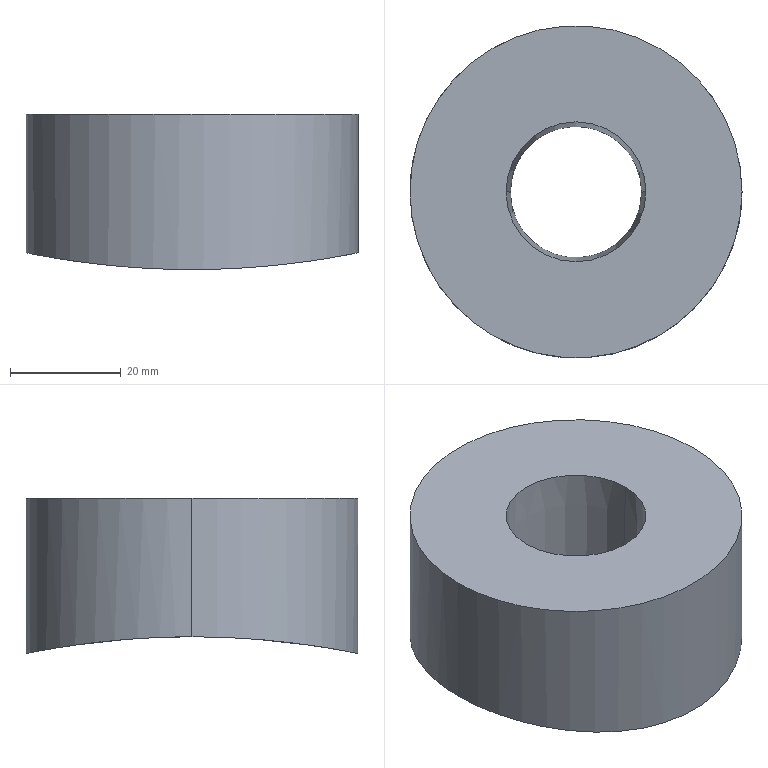Component | SolidWorks | JF21-80.1-1-3(_)-1-SOLID14-1 | 1 solid | 7 faces | box 60 x 60 x 28.03 mm | volume 60972 mm3 | cylinder 4 | cone 2 | plane 1 | commonest cylinder face diameters 300 x2 60 x2
STEP:
#1=COLOUR_RGB('',0.7922,0.8196,0.9333);
#2=FILL_AREA_STYLE_COLOUR('',#1);
#3=FILL_AREA_STYLE('',(#2));
#4=SURFACE_STYLE_FILL_AREA(#3);
#5=SURFACE_SIDE_STYLE('',(#4));
#6=SURFACE_STYLE_USAGE(.BOTH.,#5);
#7=PRESENTATION_STYLE_ASSIGNMENT((#6));
#8=CARTESIAN_POINT('',(11.417,-39.37,42.126));
#9=VERTEX_POINT('',#8);
#10=CARTESIAN_POINT('',(13.78,-39.37,42.126));
#11=VERTEX_POINT('',#10);
#12=CARTESIAN_POINT('',(11.417,-39.37,42.126));
#13=CARTESIAN_POINT('',(11.417,-39.448,42.126));
#14=CARTESIAN_POINT('',(11.425,-39.525,42.124));
#15=CARTESIAN_POINT('',(11.448,-39.639,42.12));
#16=CARTESIAN_POINT('',(11.457,-39.676,42.118));
#17=CARTESIAN_POINT('',(11.474,-39.732,42.115));
#18=CARTESIAN_POINT('',(11.48,-39.75,42.114));
#19=CARTESIAN_POINT('',(11.493,-39.787,42.111));
#20=CARTESIAN_POINT('',(11.5,-39.805,42.11));
#21=CARTESIAN_POINT('',(11.537,-39.894,42.103));
#22=CARTESIAN_POINT('',(11.574,-39.962,42.097));
#23=CARTESIAN_POINT('',(11.627,-40.042,42.088));
#24=CARTESIAN_POINT('',(11.638,-40.058,42.086));
#25=CARTESIAN_POINT('',(11.661,-40.089,42.082));
#26=CARTESIAN_POINT('',(11.673,-40.105,42.08));
#27=CARTESIAN_POINT('',(11.71,-40.15,42.074));
#28=CARTESIAN_POINT('',(11.736,-40.178,42.071));
#29=CARTESIAN_POINT('',(11.818,-40.26,42.059));
#30=CARTESIAN_POINT('',(11.877,-40.308,42.051));
#31=CARTESIAN_POINT('',(11.958,-40.362,42.042));
#32=CARTESIAN_POINT('',(11.974,-40.373,42.04));
#33=CARTESIAN_POINT('',(12.007,-40.393,42.037));
#34=CARTESIAN_POINT('',(12.024,-40.402,42.035));
#35=CARTESIAN_POINT('',(12.075,-40.43,42.03));
#36=CARTESIAN_POINT('',(12.11,-40.446,42.027));
#37=CARTESIAN_POINT('',(12.181,-40.476,42.022));
#38=CARTESIAN_POINT('',(12.217,-40.489,42.019));
#39=CARTESIAN_POINT('',(12.273,-40.506,42.016));
#40=CARTESIAN_POINT('',(12.291,-40.511,42.015));
#41=CARTESIAN_POINT('',(12.329,-40.52,42.013));
#42=CARTESIAN_POINT('',(12.348,-40.525,42.012));
#43=CARTESIAN_POINT('',(12.443,-40.544,42.008));
#44=CARTESIAN_POINT('',(12.52,-40.551,42.007));
#45=CARTESIAN_POINT('',(12.636,-40.551,42.007));
#46=CARTESIAN_POINT('',(12.675,-40.549,42.007));
#47=CARTESIAN_POINT('',(12.733,-40.544,42.008));
#48=CARTESIAN_POINT('',(12.753,-40.541,42.009));
#49=CARTESIAN_POINT('',(12.791,-40.536,42.01));
#50=CARTESIAN_POINT('',(12.81,-40.532,42.011));
#51=CARTESIAN_POINT('',(12.905,-40.513,42.014));
#52=CARTESIAN_POINT('',(12.979,-40.491,42.019));
#53=CARTESIAN_POINT('',(13.086,-40.447,42.027));
#54=CARTESIAN_POINT('',(13.121,-40.43,42.03));
#55=CARTESIAN_POINT('',(13.19,-40.393,42.037));
#56=CARTESIAN_POINT('',(13.223,-40.374,42.04));
#57=CARTESIAN_POINT('',(13.286,-40.331,42.047));
#58=CARTESIAN_POINT('',(13.317,-40.308,42.051));
#59=CARTESIAN_POINT('',(13.362,-40.271,42.057));
#60=CARTESIAN_POINT('',(13.377,-40.259,42.059));
#61=CARTESIAN_POINT('',(13.405,-40.233,42.063));
#62=CARTESIAN_POINT('',(13.419,-40.219,42.065));
#63=CARTESIAN_POINT('',(13.488,-40.151,42.074));
#64=CARTESIAN_POINT('',(13.537,-40.091,42.082));
#65=CARTESIAN_POINT('',(13.601,-39.996,42.093));
#66=CARTESIAN_POINT('',(13.621,-39.963,42.096));
#67=CARTESIAN_POINT('',(13.648,-39.911,42.101));
#68=CARTESIAN_POINT('',(13.657,-39.894,42.103));
#69=CARTESIAN_POINT('',(13.674,-39.859,42.106));
#70=CARTESIAN_POINT('',(13.682,-39.841,42.107));
#71=CARTESIAN_POINT('',(13.719,-39.752,42.114));
#72=CARTESIAN_POINT('',(13.741,-39.678,42.118));
#73=CARTESIAN_POINT('',(13.76,-39.584,42.122));
#74=CARTESIAN_POINT('',(13.764,-39.564,42.123));
#75=CARTESIAN_POINT('',(13.769,-39.526,42.124));
#76=CARTESIAN_POINT('',(13.772,-39.506,42.124));
#77=CARTESIAN_POINT('',(13.778,-39.448,42.126));
#78=CARTESIAN_POINT('',(13.78,-39.409,42.126));
#79=CARTESIAN_POINT('',(13.78,-39.37,42.126));
#80=B_SPLINE_CURVE_WITH_KNOTS('',3,(#12,#13,#14,#15,#16,#17,#18,#19,#20,#21,#22,#23,#24,#25,#26,#27,#28,#29,#30,#31,#32,#33,#34,#35,#36,#37,#38,#39,#40,#41,#42,#43,#44,#45,#46,#47,#48,#49,#50,#51,#52,#53,#54,#55,#56,#57,#58,#59,#60,#61,#62,#63,#64,#65,#66,#67,#68,#69,#70,#71,#72,#73,#74,#75,#76,#77,#78,#79),.UNSPECIFIED.,.F.,.F.,(4,2,2,2,2,2,2,2,2,2,2,2,2,2,2,2,2,2,2,2,2,2,2,2,2,2,2,2,2,2,2,2,2,4),(0.,0.005875,0.008813,0.01028,0.01175,0.01763,0.01909,0.02056,0.0235,0.02938,0.03085,0.03231,0.03525,0.03819,0.03966,0.04113,0.047,0.04994,0.05141,0.05288,0.05875,0.06169,0.06463,0.06757,0.06904,0.0705,0.07638,0.07932,0.08079,0.08226,0.08813,0.0896,0.09107,0.09401),.UNSPECIFIED.);
#81=EDGE_CURVE('',#9,#11,#80,.T.);
#82=ORIENTED_EDGE('',*,*,#81,.F.);
#83=CARTESIAN_POINT('',(12.131,-39.37,42.126));
#84=VERTEX_POINT('',#83);
#85=CARTESIAN_POINT('',(-15.748,-39.37,42.126));
#86=DIRECTION('',(1.,0.,0.));
#87=VECTOR('',#86,39.37);
#88=LINE('',#85,#87);
#89=EDGE_CURVE('',#9,#84,#88,.T.);
#90=ORIENTED_EDGE('',*,*,#89,.T.);
#91=CARTESIAN_POINT('',(13.065,-39.37,42.126));
#92=VERTEX_POINT('',#91);
#93=CARTESIAN_POINT('',(13.065,-39.37,42.126));
#94=CARTESIAN_POINT('',(13.065,-39.401,42.126));
#95=CARTESIAN_POINT('',(13.062,-39.431,42.126));
#96=CARTESIAN_POINT('',(13.053,-39.476,42.125));
#97=CARTESIAN_POINT('',(13.05,-39.491,42.125));
#98=CARTESIAN_POINT('',(13.041,-39.52,42.124));
#99=CARTESIAN_POINT('',(13.036,-39.535,42.124));
#100=CARTESIAN_POINT('',(13.018,-39.577,42.122));
#101=CARTESIAN_POINT('',(13.004,-39.604,42.121));
#102=CARTESIAN_POINT('',(12.978,-39.642,42.12));
#103=CARTESIAN_POINT('',(12.969,-39.654,42.119));
#104=CARTESIAN_POINT('',(12.95,-39.678,42.118));
#105=CARTESIAN_POINT('',(12.939,-39.689,42.117));
#106=CARTESIAN_POINT('',(12.907,-39.721,42.116));
#107=CARTESIAN_POINT('',(12.883,-39.741,42.114));
#108=CARTESIAN_POINT('',(12.845,-39.766,42.113));
#109=CARTESIAN_POINT('',(12.832,-39.774,42.112));
#110=CARTESIAN_POINT('',(12.805,-39.789,42.111));
#111=CARTESIAN_POINT('',(12.778,-39.802,42.11));
#112=CARTESIAN_POINT('',(12.749,-39.812,42.109));
#113=CARTESIAN_POINT('',(12.72,-39.821,42.109));
#114=CARTESIAN_POINT('',(12.705,-39.825,42.108));
#115=CARTESIAN_POINT('',(12.659,-39.834,42.108));
#116=CARTESIAN_POINT('',(12.629,-39.836,42.108));
#117=CARTESIAN_POINT('',(12.584,-39.837,42.108));
#118=CARTESIAN_POINT('',(12.568,-39.836,42.108));
#119=CARTESIAN_POINT('',(12.538,-39.833,42.108));
#120=CARTESIAN_POINT('',(12.522,-39.831,42.108));
#121=CARTESIAN_POINT('',(12.478,-39.822,42.109));
#122=CARTESIAN_POINT('',(12.448,-39.813,42.109));
#123=CARTESIAN_POINT('',(12.406,-39.795,42.111));
#124=CARTESIAN_POINT('',(12.392,-39.789,42.111));
#125=CARTESIAN_POINT('',(12.365,-39.774,42.112));
#126=CARTESIAN_POINT('',(12.352,-39.767,42.113));
#127=CARTESIAN_POINT('',(12.314,-39.741,42.114));
#128=CARTESIAN_POINT('',(12.29,-39.722,42.116));
#129=CARTESIAN_POINT('',(12.247,-39.678,42.118));
#130=CARTESIAN_POINT('',(12.227,-39.655,42.119));
#131=CARTESIAN_POINT('',(12.202,-39.617,42.121));
#132=CARTESIAN_POINT('',(12.194,-39.604,42.121));
#133=CARTESIAN_POINT('',(12.18,-39.577,42.122));
#134=CARTESIAN_POINT('',(12.173,-39.563,42.123));
#135=CARTESIAN_POINT('',(12.155,-39.521,42.124));
#136=CARTESIAN_POINT('',(12.147,-39.492,42.125));
#137=CARTESIAN_POINT('',(12.135,-39.432,42.126));
#138=CARTESIAN_POINT('',(12.131,-39.401,42.126));
#139=CARTESIAN_POINT('',(12.131,-39.37,42.126));
#140=B_SPLINE_CURVE_WITH_KNOTS('',3,(#93,#94,#95,#96,#97,#98,#99,#100,#101,#102,#103,#104,#105,#106,#107,#108,#109,#110,#111,#112,#113,#114,#115,#116,#117,#118,#119,#120,#121,#122,#123,#124,#125,#126,#127,#128,#129,#130,#131,#132,#133,#134,#135,#136,#137,#138,#139),.UNSPECIFIED.,.F.,.F.,(4,2,2,2,2,2,2,2,2,1,2,2,2,2,2,2,2,2,2,2,2,2,2,4),(0.,0.002317,0.003475,0.004634,0.006951,0.008109,0.009267,0.01158,0.01274,0.0139,0.01506,0.01622,0.01853,0.01969,0.02085,0.02317,0.02433,0.02549,0.0278,0.03012,0.03128,0.03244,0.03475,0.03707),.UNSPECIFIED.);
#141=EDGE_CURVE('',#92,#84,#140,.T.);
#142=ORIENTED_EDGE('',*,*,#141,.F.);
#143=CARTESIAN_POINT('',(-15.748,-39.37,42.126));
#144=DIRECTION('',(1.,0.,0.));
#145=VECTOR('',#144,39.37);
#146=LINE('',#143,#145);
#147=EDGE_CURVE('',#92,#11,#146,.T.);
#148=ORIENTED_EDGE('',*,*,#147,.T.);
#149=EDGE_LOOP('',(#82,#90,#142,#148));
#150=FACE_OUTER_BOUND('',#149,.T.);
#151=CARTESIAN_POINT('',(-15.748,-39.37,36.22));
#152=DIRECTION('',(1.,0.,0.));
#153=DIRECTION('',(0.,0.,1.));
#154=AXIS2_PLACEMENT_3D('',#151,#152,#153);
#155=CYLINDRICAL_SURFACE('',#154,5.906);
#156=ADVANCED_FACE('',(#150),#155,.F.);
#157=ORIENTED_EDGE('',*,*,#141,.T.);
#158=CARTESIAN_POINT('',(12.101,-39.37,43.11));
#159=VERTEX_POINT('',#158);
#160=CARTESIAN_POINT('',(12.101,-39.37,43.11));
#161=DIRECTION('',(-0.0312,0.,0.9995));
#162=VECTOR('',#161,39.37);
#163=LINE('',#160,#162);
#164=EDGE_CURVE('',#84,#159,#163,.T.);
#165=ORIENTED_EDGE('',*,*,#164,.T.);
#166=CARTESIAN_POINT('',(13.096,-39.37,43.11));
#167=VERTEX_POINT('',#166);
#168=CARTESIAN_POINT('',(12.598,-39.37,43.11));
#169=DIRECTION('',(0.,0.,1.));
#170=DIRECTION('',(1.,0.,0.));
#171=AXIS2_PLACEMENT_3D('',#168,#169,#170);
#172=CIRCLE('',#171,0.4977);
#173=EDGE_CURVE('',#159,#167,#172,.T.);
#174=ORIENTED_EDGE('',*,*,#173,.T.);
#175=CARTESIAN_POINT('',(13.096,-39.37,43.11));
#176=DIRECTION('',(0.0312,0.,0.9995));
#177=VECTOR('',#176,39.37);
#178=LINE('',#175,#177);
#179=EDGE_CURVE('',#92,#167,#178,.T.);
#180=ORIENTED_EDGE('',*,*,#179,.F.);
#181=EDGE_LOOP('',(#157,#165,#174,#180));
#182=FACE_OUTER_BOUND('',#181,.T.);
#183=CARTESIAN_POINT('',(12.598,-39.37,43.11));
#184=DIRECTION('',(0.,0.,1.));
#185=DIRECTION('',(-1.,0.,0.));
#186=AXIS2_PLACEMENT_3D('',#183,#184,#185);
#187=CONICAL_SURFACE('',#186,0.4977,0.03121);
#188=ADVANCED_FACE('',(#182),#187,.F.);
#189=CARTESIAN_POINT('',(13.78,-39.37,42.126));
#190=CARTESIAN_POINT('',(13.78,-39.292,42.126));
#191=CARTESIAN_POINT('',(13.772,-39.215,42.124));
#192=CARTESIAN_POINT('',(13.749,-39.102,42.12));
#193=CARTESIAN_POINT('',(13.74,-39.064,42.118));
#194=CARTESIAN_POINT('',(13.723,-39.008,42.115));
#195=CARTESIAN_POINT('',(13.717,-38.99,42.114));
#196=CARTESIAN_POINT('',(13.704,-38.953,42.111));
#197=CARTESIAN_POINT('',(13.697,-38.935,42.11));
#198=CARTESIAN_POINT('',(13.66,-38.846,42.103));
#199=CARTESIAN_POINT('',(13.623,-38.778,42.097));
#200=CARTESIAN_POINT('',(13.57,-38.698,42.088));
#201=CARTESIAN_POINT('',(13.559,-38.682,42.086));
#202=CARTESIAN_POINT('',(13.536,-38.651,42.082));
#203=CARTESIAN_POINT('',(13.524,-38.636,42.08));
#204=CARTESIAN_POINT('',(13.487,-38.591,42.074));
#205=CARTESIAN_POINT('',(13.461,-38.562,42.071));
#206=CARTESIAN_POINT('',(13.379,-38.481,42.059));
#207=CARTESIAN_POINT('',(13.32,-38.432,42.051));
#208=CARTESIAN_POINT('',(13.239,-38.378,42.042));
#209=CARTESIAN_POINT('',(13.223,-38.367,42.04));
#210=CARTESIAN_POINT('',(13.19,-38.347,42.037));
#211=CARTESIAN_POINT('',(13.173,-38.338,42.035));
#212=CARTESIAN_POINT('',(13.122,-38.311,42.03));
#213=CARTESIAN_POINT('',(13.087,-38.294,42.027));
#214=CARTESIAN_POINT('',(13.016,-38.265,42.022));
#215=CARTESIAN_POINT('',(12.98,-38.252,42.019));
#216=CARTESIAN_POINT('',(12.924,-38.235,42.016));
#217=CARTESIAN_POINT('',(12.906,-38.229,42.015));
#218=CARTESIAN_POINT('',(12.868,-38.22,42.013));
#219=CARTESIAN_POINT('',(12.849,-38.216,42.012));
#220=CARTESIAN_POINT('',(12.753,-38.197,42.008));
#221=CARTESIAN_POINT('',(12.677,-38.189,42.007));
#222=CARTESIAN_POINT('',(12.561,-38.189,42.007));
#223=CARTESIAN_POINT('',(12.522,-38.191,42.007));
#224=CARTESIAN_POINT('',(12.464,-38.197,42.008));
#225=CARTESIAN_POINT('',(12.444,-38.199,42.009));
#226=CARTESIAN_POINT('',(12.406,-38.205,42.01));
#227=CARTESIAN_POINT('',(12.387,-38.208,42.011));
#228=CARTESIAN_POINT('',(12.292,-38.227,42.014));
#229=CARTESIAN_POINT('',(12.218,-38.249,42.019));
#230=CARTESIAN_POINT('',(12.111,-38.294,42.027));
#231=CARTESIAN_POINT('',(12.076,-38.31,42.03));
#232=CARTESIAN_POINT('',(12.007,-38.347,42.037));
#233=CARTESIAN_POINT('',(11.974,-38.367,42.04));
#234=CARTESIAN_POINT('',(11.91,-38.409,42.047));
#235=CARTESIAN_POINT('',(11.88,-38.432,42.051));
#236=CARTESIAN_POINT('',(11.835,-38.469,42.057));
#237=CARTESIAN_POINT('',(11.82,-38.481,42.059));
#238=CARTESIAN_POINT('',(11.792,-38.507,42.063));
#239=CARTESIAN_POINT('',(11.777,-38.521,42.065));
#240=CARTESIAN_POINT('',(11.709,-38.589,42.074));
#241=CARTESIAN_POINT('',(11.66,-38.649,42.082));
#242=CARTESIAN_POINT('',(11.596,-38.744,42.093));
#243=CARTESIAN_POINT('',(11.576,-38.777,42.096));
#244=CARTESIAN_POINT('',(11.548,-38.829,42.101));
#245=CARTESIAN_POINT('',(11.54,-38.846,42.103));
#246=CARTESIAN_POINT('',(11.523,-38.881,42.106));
#247=CARTESIAN_POINT('',(11.515,-38.899,42.107));
#248=CARTESIAN_POINT('',(11.478,-38.988,42.114));
#249=CARTESIAN_POINT('',(11.456,-39.062,42.118));
#250=CARTESIAN_POINT('',(11.437,-39.157,42.122));
#251=CARTESIAN_POINT('',(11.433,-39.176,42.123));
#252=CARTESIAN_POINT('',(11.427,-39.214,42.124));
#253=CARTESIAN_POINT('',(11.425,-39.234,42.124));
#254=CARTESIAN_POINT('',(11.419,-39.292,42.126));
#255=CARTESIAN_POINT('',(11.417,-39.331,42.126));
#256=CARTESIAN_POINT('',(11.417,-39.37,42.126));
#257=B_SPLINE_CURVE_WITH_KNOTS('',3,(#189,#190,#191,#192,#193,#194,#195,#196,#197,#198,#199,#200,#201,#202,#203,#204,#205,#206,#207,#208,#209,#210,#211,#212,#213,#214,#215,#216,#217,#218,#219,#220,#221,#222,#223,#224,#225,#226,#227,#228,#229,#230,#231,#232,#233,#234,#235,#236,#237,#238,#239,#240,#241,#242,#243,#244,#245,#246,#247,#248,#249,#250,#251,#252,#253,#254,#255,#256),.UNSPECIFIED.,.F.,.F.,(4,2,2,2,2,2,2,2,2,2,2,2,2,2,2,2,2,2,2,2,2,2,2,2,2,2,2,2,2,2,2,2,2,4),(0.,0.005875,0.008813,0.01028,0.01175,0.01763,0.01909,0.02056,0.0235,0.02938,0.03085,0.03231,0.03525,0.03819,0.03966,0.04113,0.047,0.04994,0.05141,0.05288,0.05875,0.06169,0.06463,0.06757,0.06904,0.0705,0.07638,0.07932,0.08079,0.08226,0.08813,0.0896,0.09107,0.09401),.UNSPECIFIED.);
#258=EDGE_CURVE('',#11,#9,#257,.T.);
#259=ORIENTED_EDGE('',*,*,#258,.T.);
#260=CARTESIAN_POINT('',(11.417,-39.37,43.11));
#261=VERTEX_POINT('',#260);
#262=CARTESIAN_POINT('',(11.417,-39.37,41.929));
#263=DIRECTION('',(0.,0.,1.));
#264=VECTOR('',#263,39.37);
#265=LINE('',#262,#264);
#266=EDGE_CURVE('',#9,#261,#265,.T.);
#267=ORIENTED_EDGE('',*,*,#266,.T.);
#268=CARTESIAN_POINT('',(13.78,-39.37,43.11));
#269=VERTEX_POINT('',#268);
#270=CARTESIAN_POINT('',(12.598,-39.37,43.11));
#271=DIRECTION('',(0.,0.,1.));
#272=DIRECTION('',(1.,0.,0.));
#273=AXIS2_PLACEMENT_3D('',#270,#271,#272);
#274=CIRCLE('',#273,1.181);
#275=EDGE_CURVE('',#269,#261,#274,.T.);
#276=ORIENTED_EDGE('',*,*,#275,.F.);
#277=CARTESIAN_POINT('',(13.78,-39.37,41.929));
#278=DIRECTION('',(0.,0.,1.));
#279=VECTOR('',#278,39.37);
#280=LINE('',#277,#279);
#281=EDGE_CURVE('',#11,#269,#280,.T.);
#282=ORIENTED_EDGE('',*,*,#281,.F.);
#283=EDGE_LOOP('',(#259,#267,#276,#282));
#284=FACE_OUTER_BOUND('',#283,.T.);
#285=CARTESIAN_POINT('',(12.598,-39.37,41.929));
#286=DIRECTION('',(0.,0.,1.));
#287=DIRECTION('',(-1.,0.,0.));
#288=AXIS2_PLACEMENT_3D('',#285,#286,#287);
#289=CYLINDRICAL_SURFACE('',#288,1.181);
#290=ADVANCED_FACE('',(#284),#289,.T.);
#291=ORIENTED_EDGE('',*,*,#266,.F.);
#292=ORIENTED_EDGE('',*,*,#81,.T.);
#293=ORIENTED_EDGE('',*,*,#281,.T.);
#294=CARTESIAN_POINT('',(12.598,-39.37,43.11));
#295=DIRECTION('',(0.,0.,1.));
#296=DIRECTION('',(1.,0.,0.));
#297=AXIS2_PLACEMENT_3D('',#294,#295,#296);
#298=CIRCLE('',#297,1.181);
#299=EDGE_CURVE('',#261,#269,#298,.T.);
#300=ORIENTED_EDGE('',*,*,#299,.F.);
#301=EDGE_LOOP('',(#291,#292,#293,#300));
#302=FACE_OUTER_BOUND('',#301,.T.);
#303=CARTESIAN_POINT('',(12.598,-39.37,41.929));
#304=DIRECTION('',(0.,0.,1.));
#305=DIRECTION('',(-1.,0.,0.));
#306=AXIS2_PLACEMENT_3D('',#303,#304,#305);
#307=CYLINDRICAL_SURFACE('',#306,1.181);
#308=ADVANCED_FACE('',(#302),#307,.T.);
#309=CARTESIAN_POINT('',(12.598,-39.37,43.11));
#310=DIRECTION('',(0.,0.,1.));
#311=DIRECTION('',(1.,0.,0.));
#312=AXIS2_PLACEMENT_3D('',#309,#310,#311);
#313=CIRCLE('',#312,0.4977);
#314=EDGE_CURVE('',#167,#159,#313,.T.);
#315=ORIENTED_EDGE('',*,*,#314,.F.);
#316=ORIENTED_EDGE('',*,*,#173,.F.);
#317=EDGE_LOOP('',(#315,#316));
#318=FACE_BOUND('',#317,.T.);
#319=ORIENTED_EDGE('',*,*,#275,.T.);
#320=ORIENTED_EDGE('',*,*,#299,.T.);
#321=EDGE_LOOP('',(#319,#320));
#322=FACE_OUTER_BOUND('',#321,.T.);
#323=CARTESIAN_POINT('',(12.598,-39.37,43.11));
#324=DIRECTION('',(0.,0.,1.));
#325=DIRECTION('',(-1.,0.,0.));
#326=AXIS2_PLACEMENT_3D('',#323,#324,#325);
#327=PLANE('',#326);
#328=ADVANCED_FACE('',(#318,#322),#327,.T.);
#329=ORIENTED_EDGE('',*,*,#89,.F.);
#330=ORIENTED_EDGE('',*,*,#258,.F.);
#331=ORIENTED_EDGE('',*,*,#147,.F.);
#332=CARTESIAN_POINT('',(12.131,-39.37,42.126));
#333=CARTESIAN_POINT('',(12.131,-39.339,42.126));
#334=CARTESIAN_POINT('',(12.134,-39.309,42.126));
#335=CARTESIAN_POINT('',(12.143,-39.264,42.125));
#336=CARTESIAN_POINT('',(12.147,-39.249,42.125));
#337=CARTESIAN_POINT('',(12.156,-39.22,42.124));
#338=CARTESIAN_POINT('',(12.161,-39.205,42.124));
#339=CARTESIAN_POINT('',(12.179,-39.163,42.122));
#340=CARTESIAN_POINT('',(12.193,-39.136,42.121));
#341=CARTESIAN_POINT('',(12.219,-39.098,42.12));
#342=CARTESIAN_POINT('',(12.228,-39.086,42.119));
#343=CARTESIAN_POINT('',(12.247,-39.062,42.118));
#344=CARTESIAN_POINT('',(12.258,-39.051,42.117));
#345=CARTESIAN_POINT('',(12.29,-39.019,42.116));
#346=CARTESIAN_POINT('',(12.313,-38.999,42.114));
#347=CARTESIAN_POINT('',(12.352,-38.974,42.113));
#348=CARTESIAN_POINT('',(12.365,-38.966,42.112));
#349=CARTESIAN_POINT('',(12.392,-38.951,42.111));
#350=CARTESIAN_POINT('',(12.419,-38.939,42.11));
#351=CARTESIAN_POINT('',(12.448,-38.928,42.109));
#352=CARTESIAN_POINT('',(12.477,-38.919,42.109));
#353=CARTESIAN_POINT('',(12.492,-38.916,42.108));
#354=CARTESIAN_POINT('',(12.537,-38.907,42.108));
#355=CARTESIAN_POINT('',(12.568,-38.904,42.108));
#356=CARTESIAN_POINT('',(12.613,-38.904,42.108));
#357=CARTESIAN_POINT('',(12.629,-38.904,42.108));
#358=CARTESIAN_POINT('',(12.659,-38.907,42.108));
#359=CARTESIAN_POINT('',(12.674,-38.91,42.108));
#360=CARTESIAN_POINT('',(12.719,-38.919,42.109));
#361=CARTESIAN_POINT('',(12.748,-38.927,42.109));
#362=CARTESIAN_POINT('',(12.791,-38.945,42.111));
#363=CARTESIAN_POINT('',(12.805,-38.951,42.111));
#364=CARTESIAN_POINT('',(12.832,-38.966,42.112));
#365=CARTESIAN_POINT('',(12.845,-38.974,42.113));
#366=CARTESIAN_POINT('',(12.883,-38.999,42.114));
#367=CARTESIAN_POINT('',(12.906,-39.018,42.116));
#368=CARTESIAN_POINT('',(12.95,-39.062,42.118));
#369=CARTESIAN_POINT('',(12.969,-39.085,42.119));
#370=CARTESIAN_POINT('',(12.995,-39.123,42.121));
#371=CARTESIAN_POINT('',(13.003,-39.136,42.121));
#372=CARTESIAN_POINT('',(13.017,-39.163,42.122));
#373=CARTESIAN_POINT('',(13.024,-39.177,42.123));
#374=CARTESIAN_POINT('',(13.041,-39.219,42.124));
#375=CARTESIAN_POINT('',(13.05,-39.249,42.125));
#376=CARTESIAN_POINT('',(13.062,-39.308,42.126));
#377=CARTESIAN_POINT('',(13.065,-39.339,42.126));
#378=CARTESIAN_POINT('',(13.065,-39.37,42.126));
#379=B_SPLINE_CURVE_WITH_KNOTS('',3,(#332,#333,#334,#335,#336,#337,#338,#339,#340,#341,#342,#343,#344,#345,#346,#347,#348,#349,#350,#351,#352,#353,#354,#355,#356,#357,#358,#359,#360,#361,#362,#363,#364,#365,#366,#367,#368,#369,#370,#371,#372,#373,#374,#375,#376,#377,#378),.UNSPECIFIED.,.F.,.F.,(4,2,2,2,2,2,2,2,2,1,2,2,2,2,2,2,2,2,2,2,2,2,2,4),(0.,0.002317,0.003475,0.004634,0.006951,0.008109,0.009267,0.01158,0.01274,0.0139,0.01506,0.01622,0.01853,0.01969,0.02085,0.02317,0.02433,0.02549,0.0278,0.03012,0.03128,0.03244,0.03475,0.03707),.UNSPECIFIED.);
#380=EDGE_CURVE('',#84,#92,#379,.T.);
#381=ORIENTED_EDGE('',*,*,#380,.F.);
#382=EDGE_LOOP('',(#329,#330,#331,#381));
#383=FACE_OUTER_BOUND('',#382,.T.);
#384=CARTESIAN_POINT('',(-15.748,-39.37,36.22));
#385=DIRECTION('',(1.,0.,0.));
#386=DIRECTION('',(0.,0.,1.));
#387=AXIS2_PLACEMENT_3D('',#384,#385,#386);
#388=CYLINDRICAL_SURFACE('',#387,5.906);
#389=ADVANCED_FACE('',(#383),#388,.F.);
#390=ORIENTED_EDGE('',*,*,#164,.F.);
#391=ORIENTED_EDGE('',*,*,#380,.T.);
#392=ORIENTED_EDGE('',*,*,#179,.T.);
#393=ORIENTED_EDGE('',*,*,#314,.T.);
#394=EDGE_LOOP('',(#390,#391,#392,#393));
#395=FACE_OUTER_BOUND('',#394,.T.);
#396=CARTESIAN_POINT('',(12.598,-39.37,43.11));
#397=DIRECTION('',(0.,0.,1.));
#398=DIRECTION('',(-1.,0.,0.));
#399=AXIS2_PLACEMENT_3D('',#396,#397,#398);
#400=CONICAL_SURFACE('',#399,0.4977,0.03121);
#401=ADVANCED_FACE('',(#395),#400,.F.);
#402=CLOSED_SHELL('',(#156,#188,#290,#308,#328,#389,#401));
#403=MANIFOLD_SOLID_BREP('',#402);
#404=STYLED_ITEM('',(#7),#403);
#405=PRESENTATION_LAYER_ASSIGNMENT('','',(#404));
#406=(LENGTH_UNIT()NAMED_UNIT(*)SI_UNIT($,.METRE.));
#407=LENGTH_MEASURE_WITH_UNIT(LENGTH_MEASURE(0.0254),#406);
#408=DIMENSIONAL_EXPONENTS(1.,0.,0.,0.,0.,0.,0.);
#409=(CONVERSION_BASED_UNIT('',#407)LENGTH_UNIT()NAMED_UNIT(#408));
#410=UNCERTAINTY_MEASURE_WITH_UNIT(LENGTH_MEASURE(0.00001),#409,'','');
#411=(NAMED_UNIT(*)PLANE_ANGLE_UNIT()SI_UNIT($,.RADIAN.));
#412=(NAMED_UNIT(*)SI_UNIT($,.STERADIAN.)SOLID_ANGLE_UNIT());
#413=(GEOMETRIC_REPRESENTATION_CONTEXT(3)GLOBAL_UNCERTAINTY_ASSIGNED_CONTEXT((#410))GLOBAL_UNIT_ASSIGNED_CONTEXT((#409,#411,#412))REPRESENTATION_CONTEXT('',''));
#414=MECHANICAL_DESIGN_GEOMETRIC_PRESENTATION_REPRESENTATION('',(#404),#413);
#415=CARTESIAN_POINT('',(0.,0.,0.));
#416=DIRECTION('',(0.,0.,1.));
#417=DIRECTION('',(1.,0.,0.));
#418=AXIS2_PLACEMENT_3D('',#415,#416,#417);
#419=(LENGTH_UNIT()NAMED_UNIT(*)SI_UNIT($,.METRE.));
#420=LENGTH_MEASURE_WITH_UNIT(LENGTH_MEASURE(0.0254),#419);
#421=DIMENSIONAL_EXPONENTS(1.,0.,0.,0.,0.,0.,0.);
#422=(CONVERSION_BASED_UNIT('',#420)LENGTH_UNIT()NAMED_UNIT(#421));
#423=UNCERTAINTY_MEASURE_WITH_UNIT(LENGTH_MEASURE(0.00001),#422,'','');
#424=(NAMED_UNIT(*)PLANE_ANGLE_UNIT()SI_UNIT($,.RADIAN.));
#425=(NAMED_UNIT(*)SI_UNIT($,.STERADIAN.)SOLID_ANGLE_UNIT());
#426=(GEOMETRIC_REPRESENTATION_CONTEXT(3)GLOBAL_UNCERTAINTY_ASSIGNED_CONTEXT((#423))GLOBAL_UNIT_ASSIGNED_CONTEXT((#422,#424,#425))REPRESENTATION_CONTEXT('',''));
#427=ADVANCED_BREP_SHAPE_REPRESENTATION('',(#403,#418),#426);